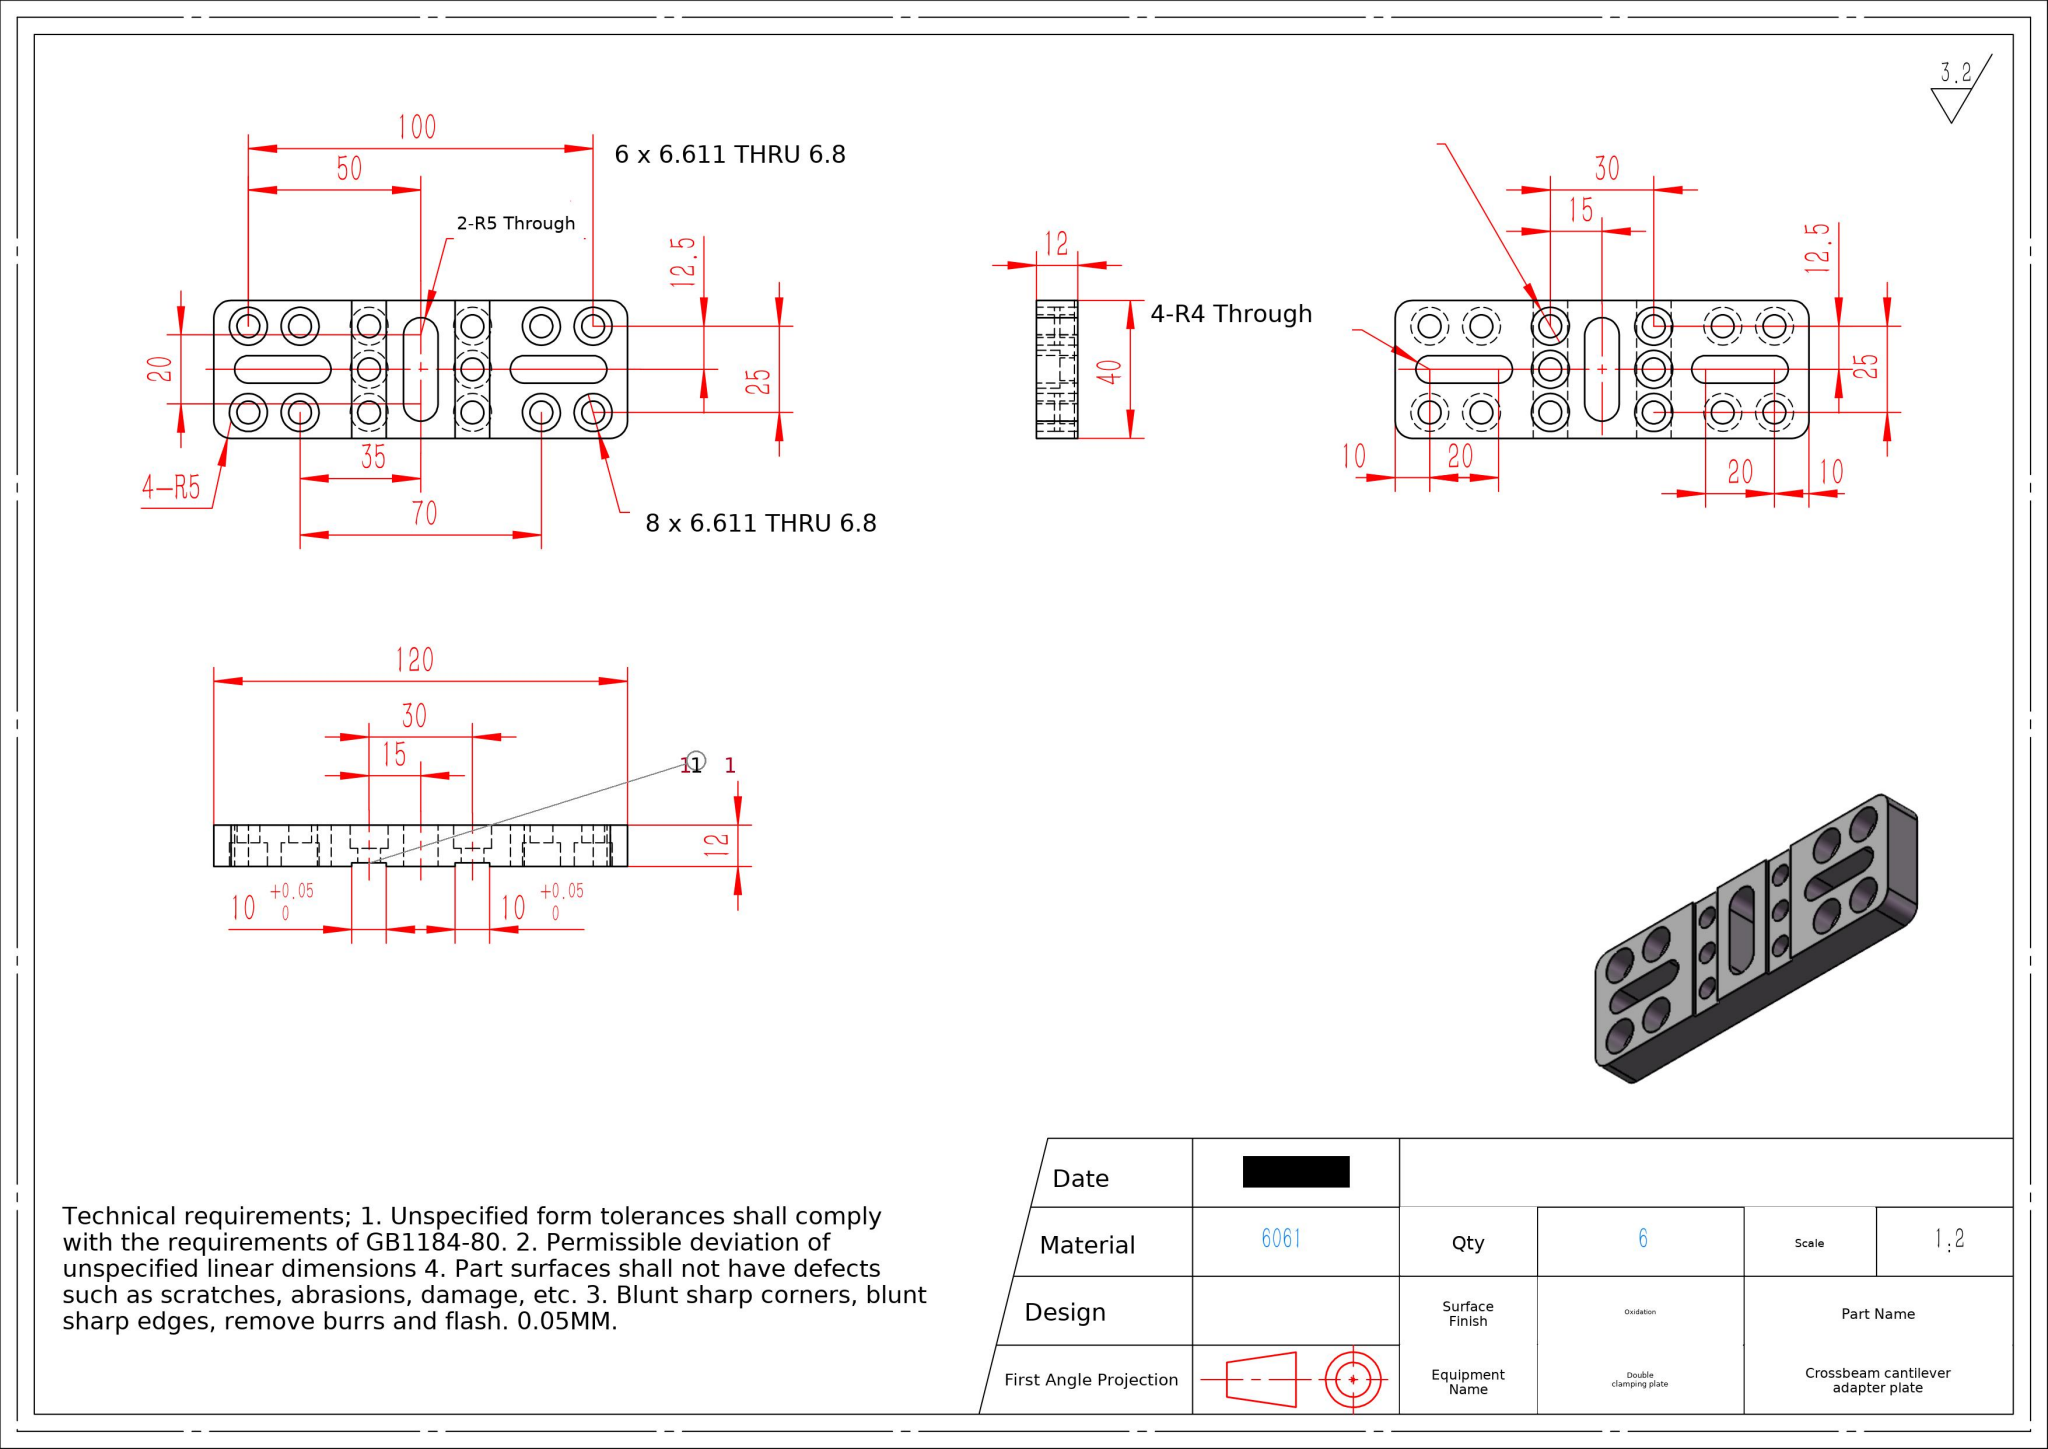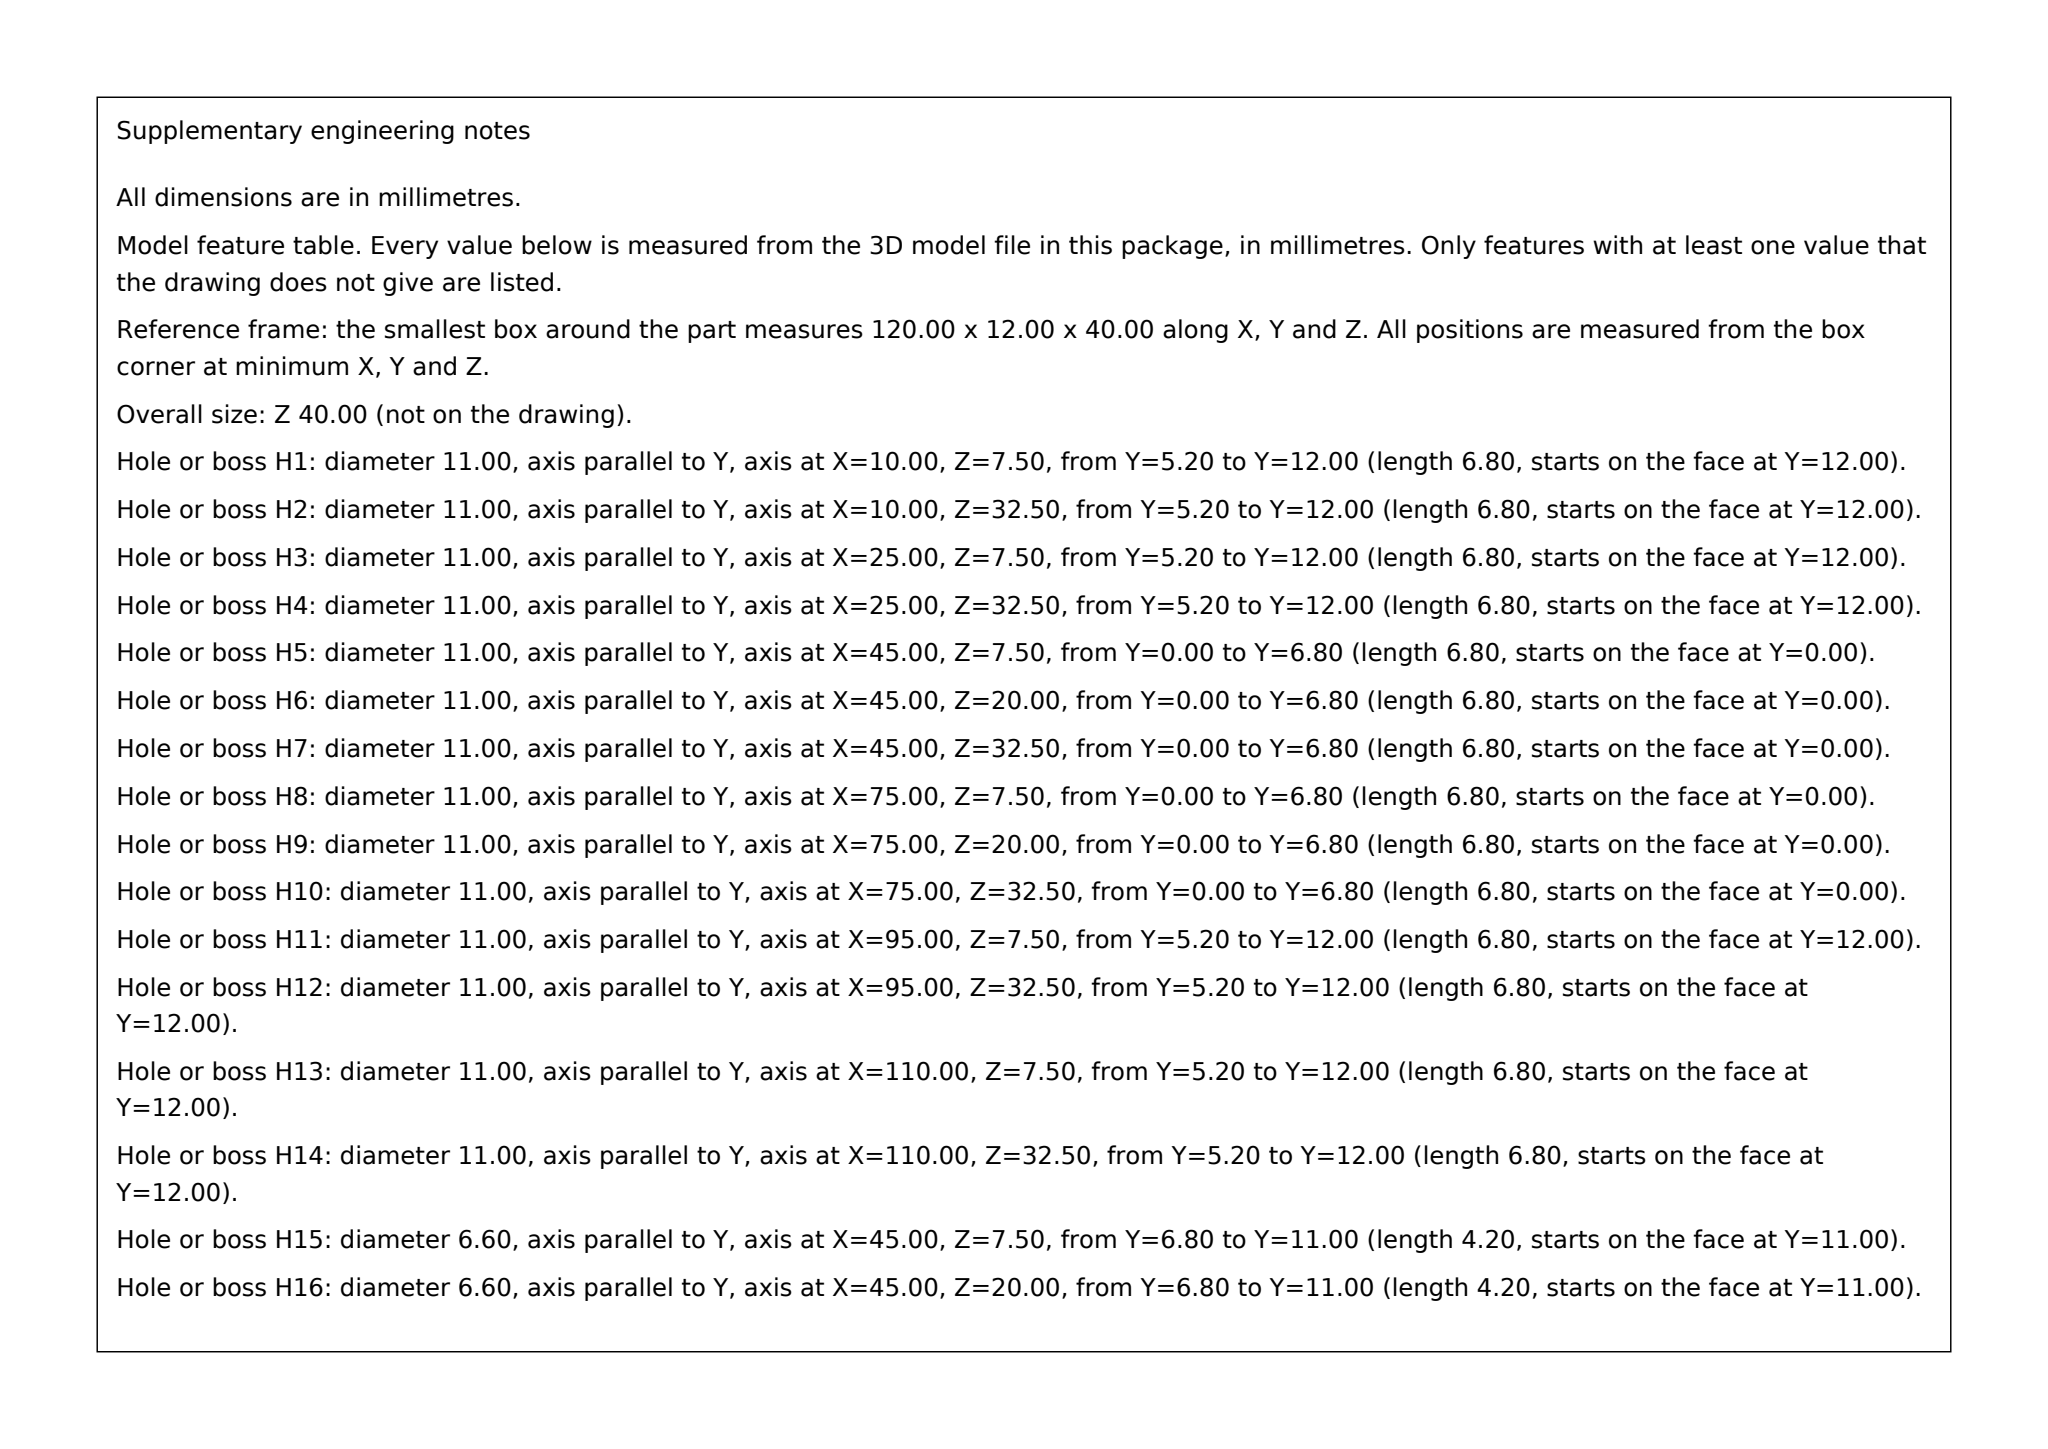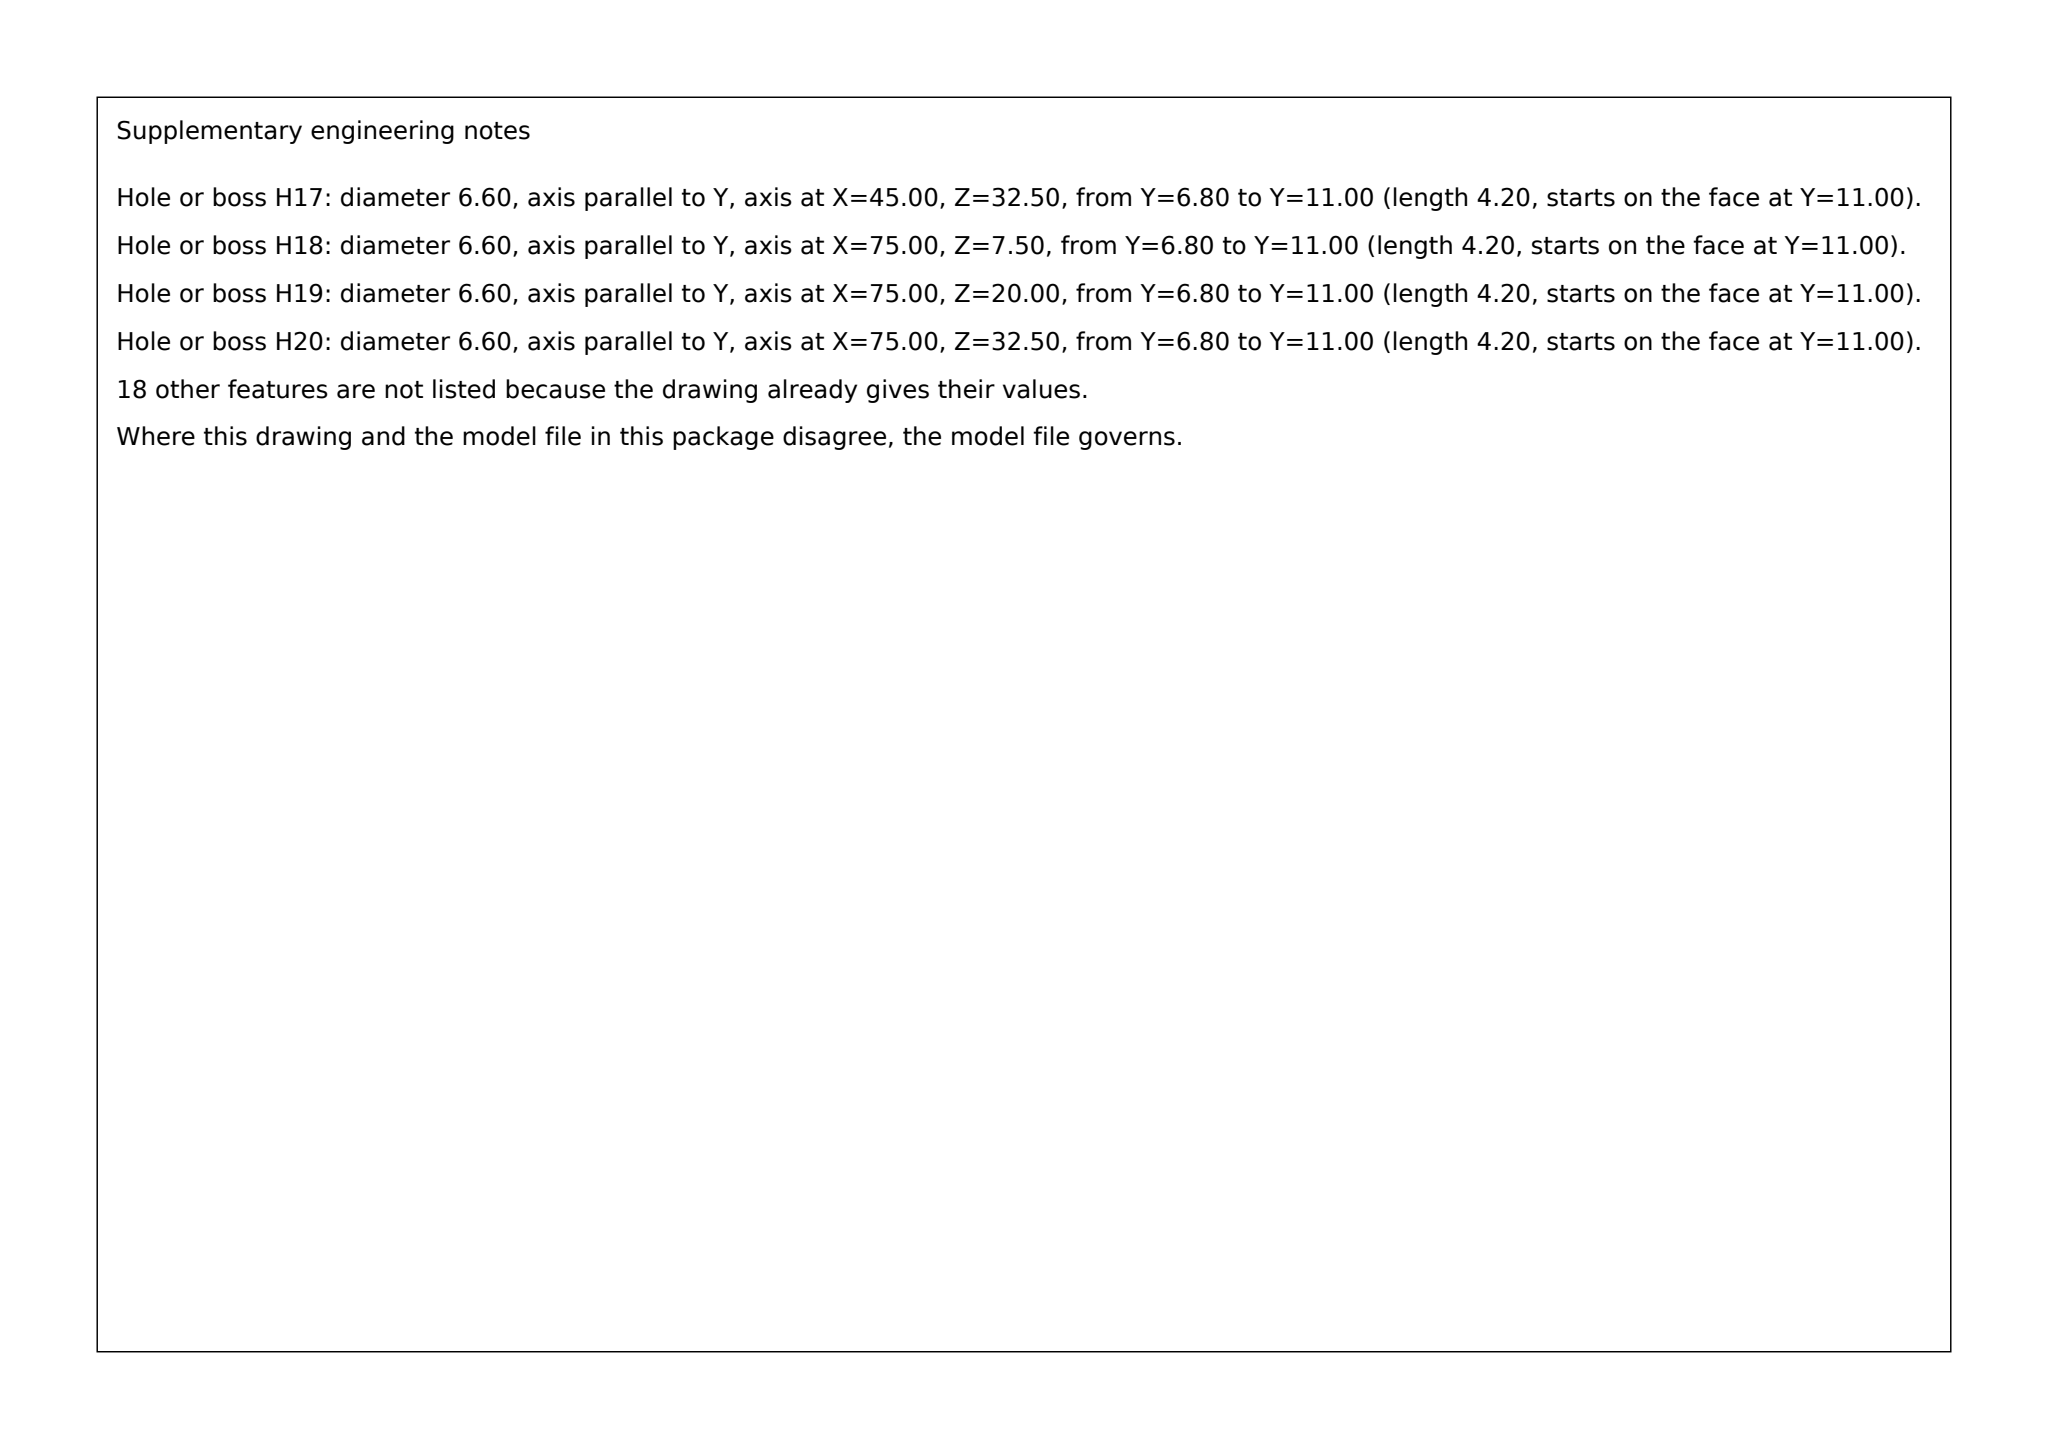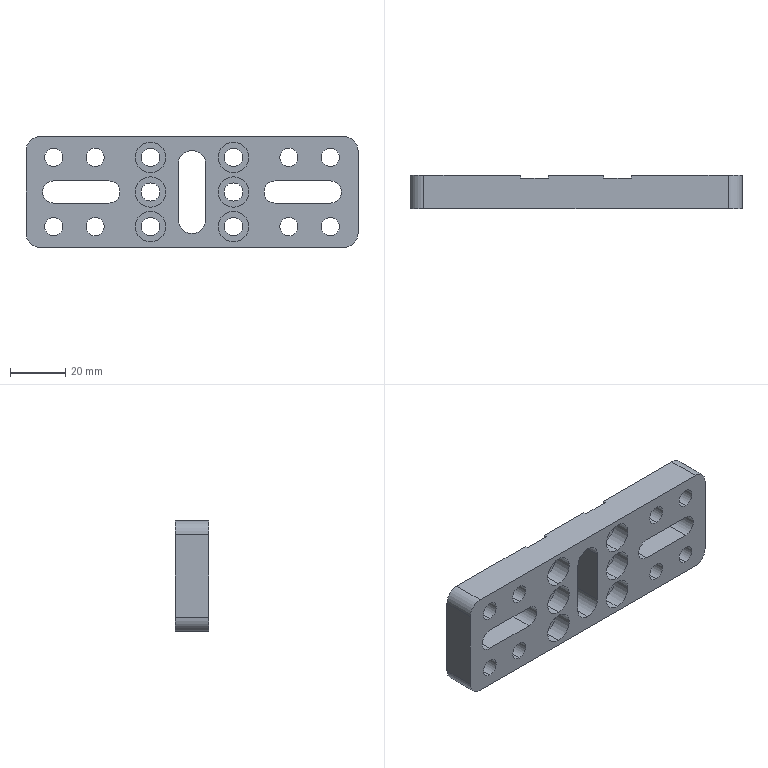Part | SolidWorks | mm | material 6061 | 1 solid | 101 faces | box 120 x 12 x 40 mm | volume 36821 mm3 | cylinder 67 | plane 34 | commonest cylinder face diameters 11 x28 6.6 x28 10 x7 8 x4
build123d program:
from build123d import *

# Parameters (mm, degrees)
SKETCH1_W                                           = 120
SKETCH1_H                                           = 40
BOSS_EXTRUDE1_DEPTH                                 = 12
SKETCH2_W                                           = 10
SKETCH2_H                                           = 1
CUT_EXTRUDE1_DEPTH                                  = 74.103
CUT_EXTRUDE4_DEPTH                                  = 65.374
CUT_EXTRUDE5_DEPTH                                  = 65.374
CYLINDRICAL_COUNTERSUNK_HOLE_FOR_M6_HEX_D           = 6.6
CYLINDRICAL_COUNTERSUNK_HOLE_FOR_M6_HEX_CBORE_D     = 11
CYLINDRICAL_COUNTERSUNK_HOLE_FOR_M6_HEX_CBORE_DEPTH = 6.8
CYLINDRICAL_COUNTERSUNK_HOLE_FOR_M6_2_D             = 6.6
CYLINDRICAL_COUNTERSUNK_HOLE_FOR_M6_2_CBORE_D       = 11
CYLINDRICAL_COUNTERSUNK_HOLE_FOR_M6_2_CBORE_DEPTH   = 6.8
FILLET1_R                                           = 5


with BuildPart() as part:
    # Sketch1 → Boss-Extrude1 (new body)
    with BuildSketch(Plane.XZ):
        Rectangle(SKETCH1_W, SKETCH1_H)
    extrude(amount=-BOSS_EXTRUDE1_DEPTH)

    # Sketch2 → Cut-Extrude1 (cut, through all)
    with BuildSketch(Plane.XY.offset(20)):
        with Locations((-15, 11.5)):
            Rectangle(SKETCH2_W, SKETCH2_H)
    cut_extrude1 = extrude(amount=-CUT_EXTRUDE1_DEPTH, mode=Mode.SUBTRACT)

    # Sketch5 → Cut-Extrude4 (cut, through all)
    with BuildSketch(Plane.XZ):
        with BuildLine():
            Line((-5, 10), (-5, -10))
            ThreePointArc((-5, -10), (0, -15), (5, -10))
            Line((5, -10), (5, 10))
            ThreePointArc((5, 10), (0, 15), (-5, 10))
        make_face()
    extrude(amount=-CUT_EXTRUDE4_DEPTH, mode=Mode.SUBTRACT)

    # Sketch6 → Cut-Extrude5 (cut, through all)
    with BuildSketch(Plane(origin=(0, 12, 0), x_dir=(-1, 0, 0), z_dir=(0, 1, 0))):
        with BuildLine():
            Line((50, 4), (30, 4))
            ThreePointArc((30, 4), (26, 0), (30, -4))
            Line((30, -4), (50, -4))
            ThreePointArc((50, -4), (54, 0), (50, 4))
        make_face()
    cut_extrude5 = extrude(amount=-CUT_EXTRUDE5_DEPTH, mode=Mode.SUBTRACT)

    # Cylindrical Countersunk Hole for M6 Hex (through all)
    with Locations(Plane(origin=(0, 12, 0), x_dir=(1, 0, 0), z_dir=(0, 1, 0))):
        with Locations((-50, 12.5), (-35, 12.5), (-35, -12.5), (-50, -12.5), (35, -12.5), (50, -12.5), (50, 12.5), (35, 12.5)):
            CounterBoreHole(CYLINDRICAL_COUNTERSUNK_HOLE_FOR_M6_HEX_D / 2, CYLINDRICAL_COUNTERSUNK_HOLE_FOR_M6_HEX_CBORE_D / 2, CYLINDRICAL_COUNTERSUNK_HOLE_FOR_M6_HEX_CBORE_DEPTH)

    # Cylindrical Countersunk Hole for M6  2 (through all)
    with Locations(Plane(origin=(0, 0, 0), x_dir=(-1, 0, 0), z_dir=(0, -1, 0))):
        with Locations((-15, 0), (15, 0), (-15, 12.5), (15, 12.5), (15, -12.5), (-15, -12.5)):
            CounterBoreHole(CYLINDRICAL_COUNTERSUNK_HOLE_FOR_M6_2_D / 2, CYLINDRICAL_COUNTERSUNK_HOLE_FOR_M6_2_CBORE_D / 2, CYLINDRICAL_COUNTERSUNK_HOLE_FOR_M6_2_CBORE_DEPTH)

    # Fillet1
    fillet1_edges = [part.edges().sort_by_distance(p)[0] for p in [
        (60, 6, 20),
        (60, 6, -20),
        (-60, 6, -20),
        (-60, 6, 20),
    ]]
    fillet(fillet1_edges, radius=FILLET1_R)

    # Mirror1: Cut-Extrude1, Cut-Extrude5 across plane
    add(cut_extrude1.mirror(Plane(origin=(0, 0, 0), x_dir=(0, 0, 1), z_dir=(1, 0, 0))), mode=Mode.SUBTRACT)
    add(cut_extrude5.mirror(Plane(origin=(0, 0, 0), x_dir=(0, 0, 1), z_dir=(1, 0, 0))), mode=Mode.SUBTRACT)


solid = part.part